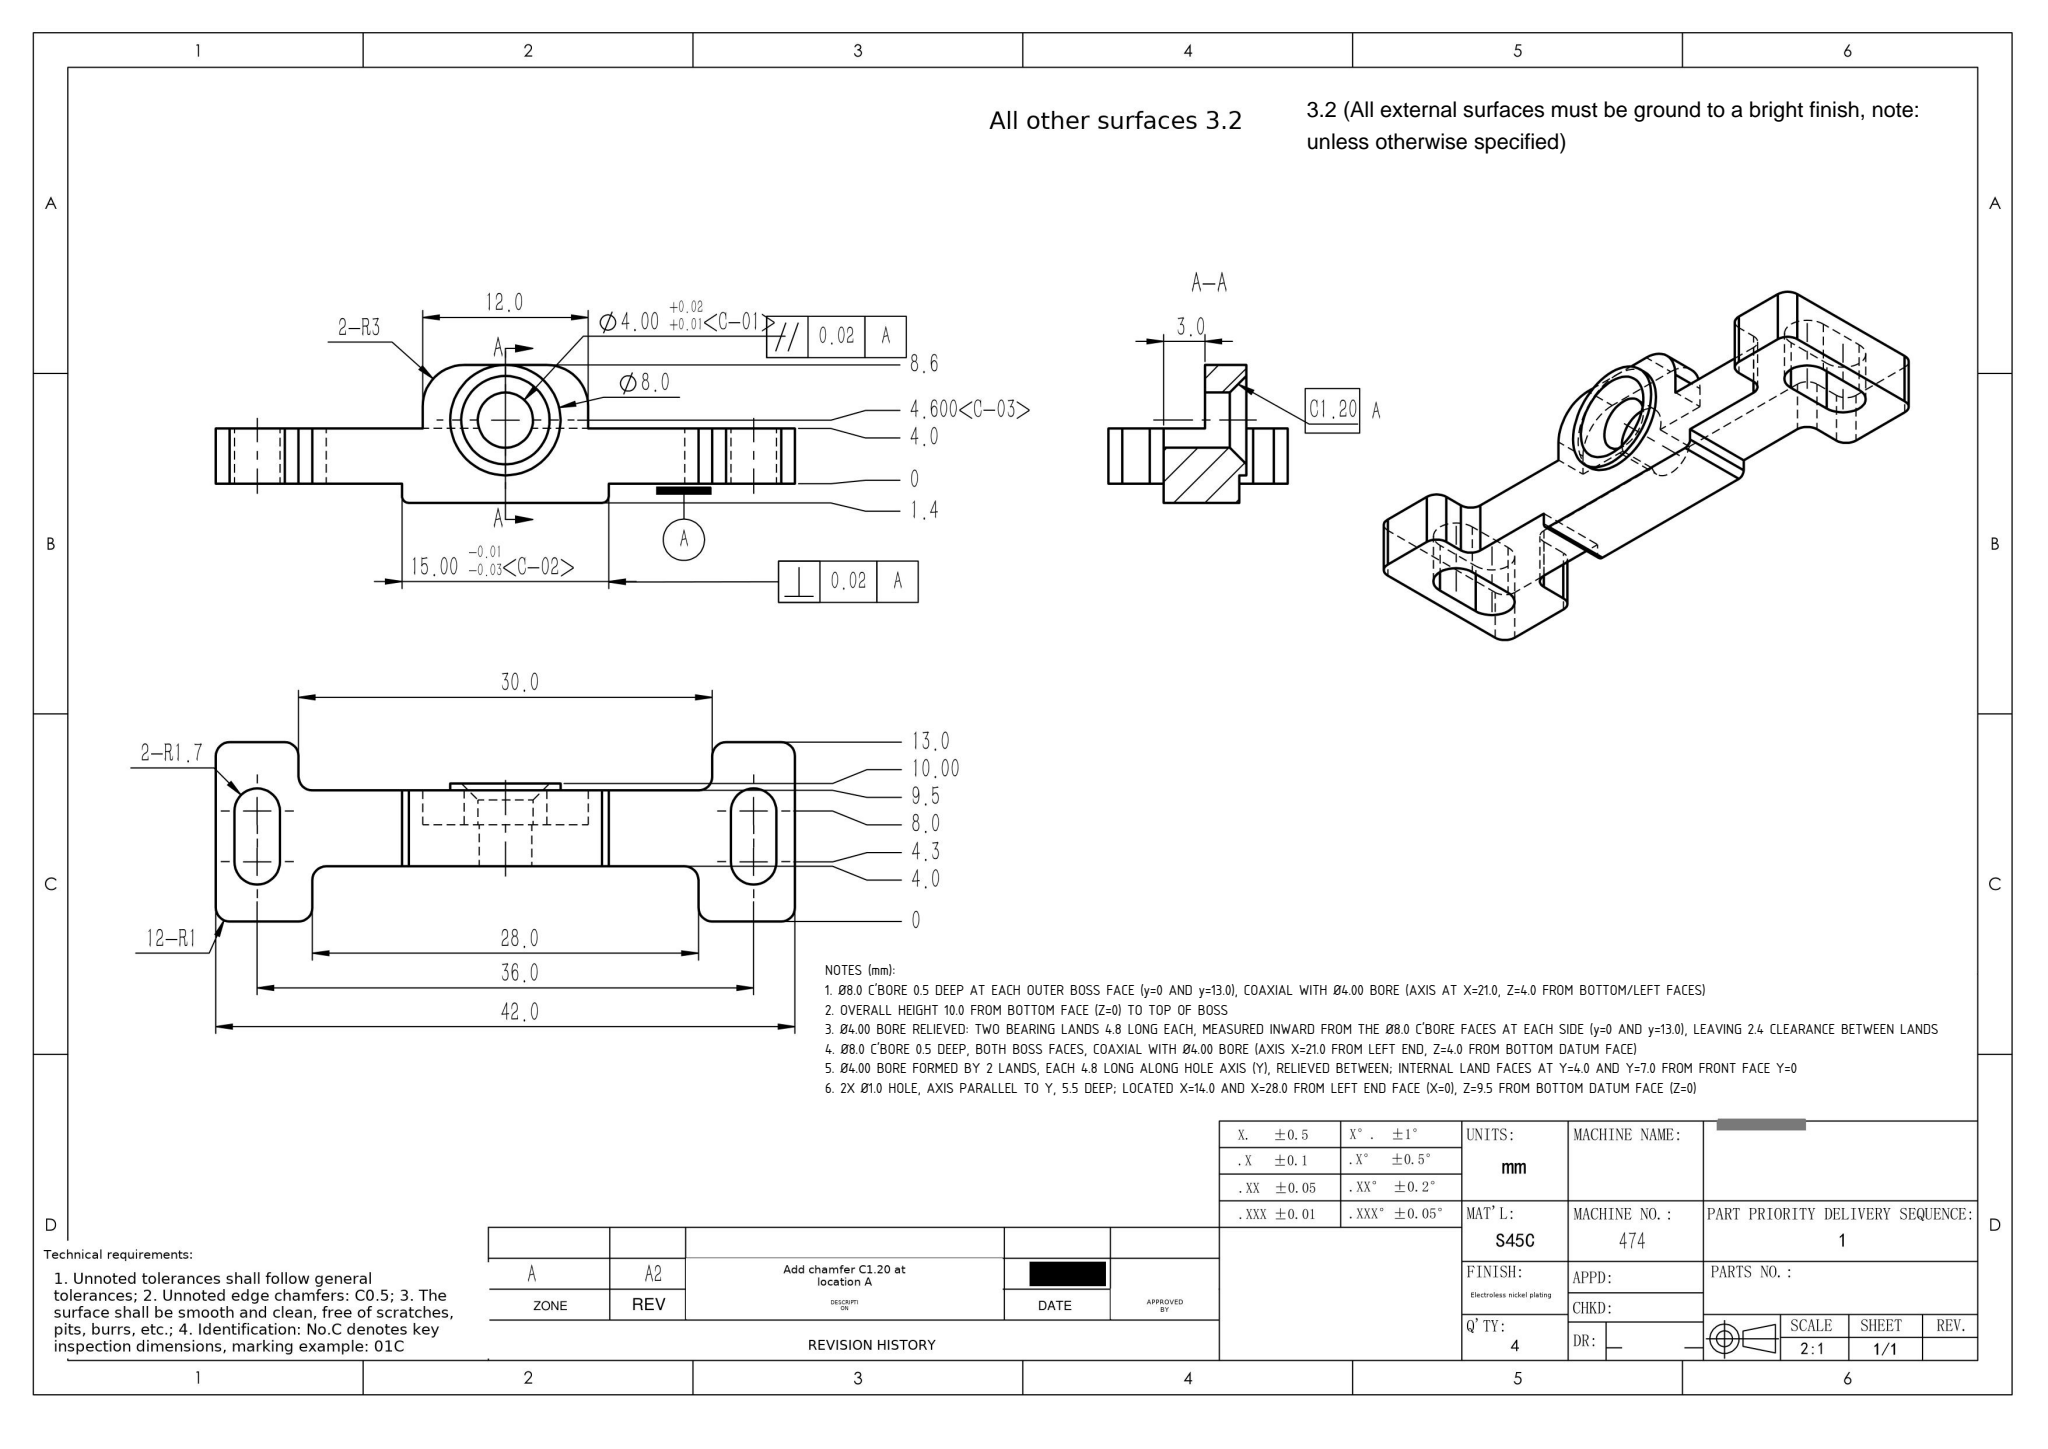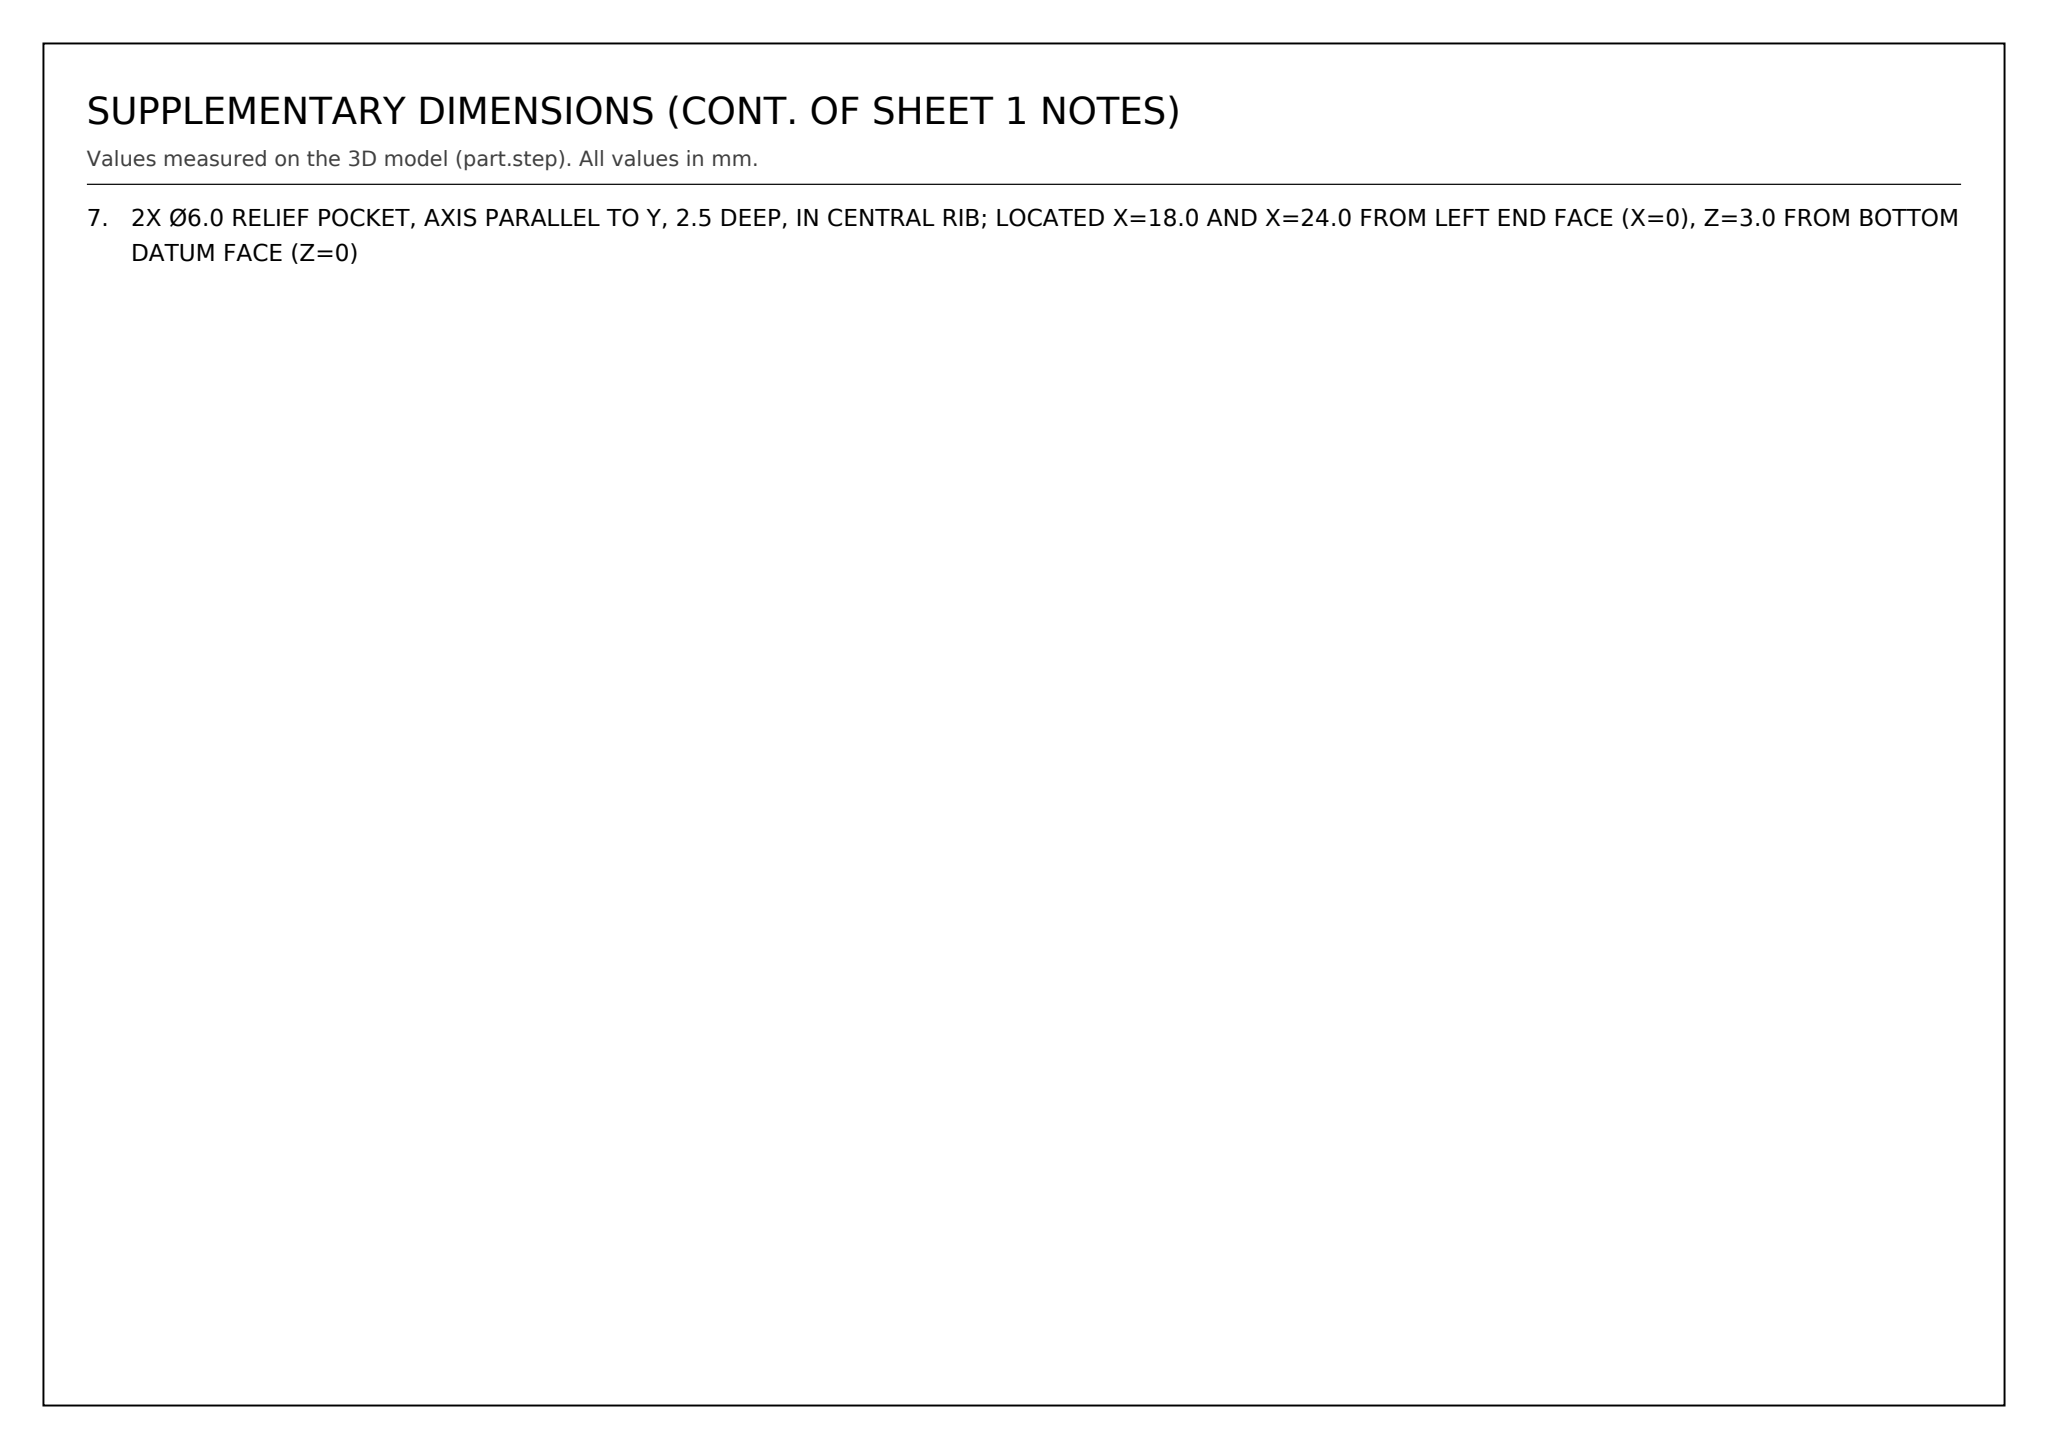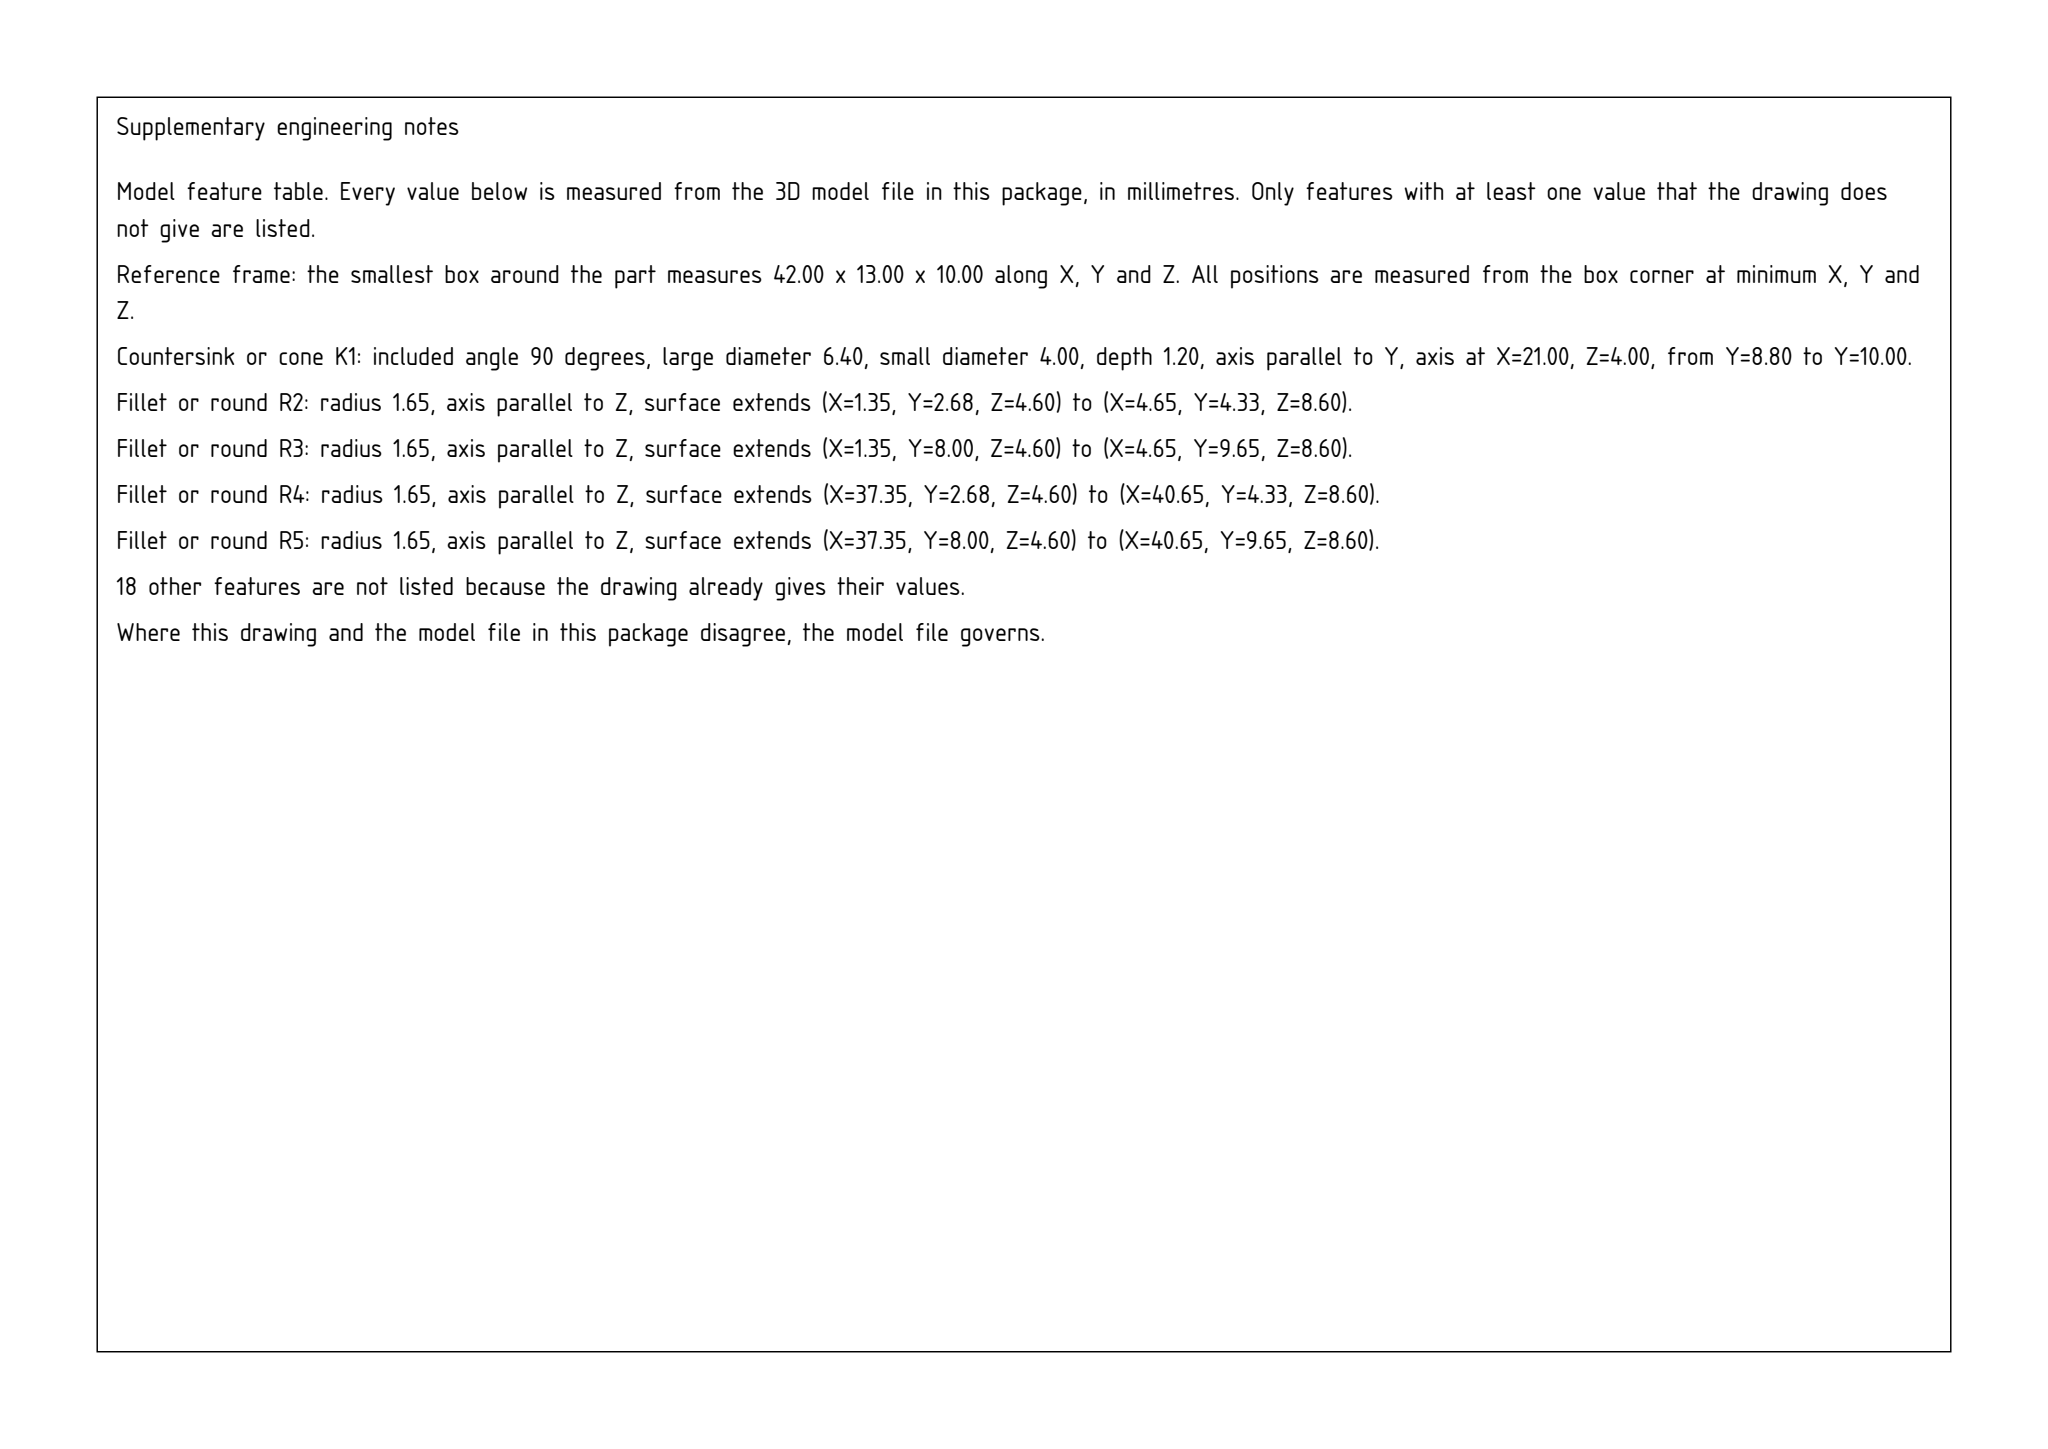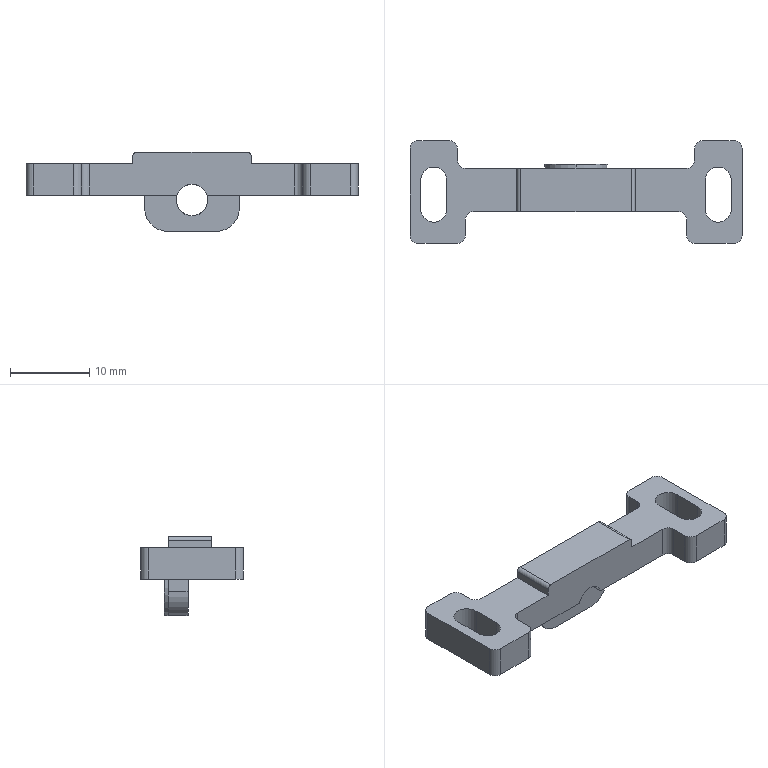Part | SolidWorks | mm | 1 solid | 54 faces | box 42 x 13 x 10 mm | volume 1355 mm3 | plane 28 | cylinder 24 | cone 2 | commonest cylinder face diameters 2 x12 3.3 x4 8 x2 4 x2 6 x2 1 x2
Drawing notes:
Ø8.0 C'BORE 0.5 DEEP AT EACH OUTER BOSS FACE (y=0 AND y=13.0), COAXIAL WITH Ø4.00 BORE (AXIS AT X=21.0, Z=4.0 FROM BOTTOM/LEFT FACES) | from the solid: cylinders: [8.0,"y",[21.0,null,4.0],0.5,count 2]
OVERALL HEIGHT 10.0 FROM BOTTOM FACE (Z=0) TO TOP OF BOSS | from the solid: bbox_xyz z = 10.0; axis_plane ["z",10.0]
Ø4.00 BORE RELIEVED: TWO BEARING LANDS 4.8 LONG EACH, MEASURED INWARD FROM THE Ø8.0 C'BORE FACES AT EACH SIDE (y=0 AND y=13.0), LEAVING 2.4 CLEARANCE BETWEEN LANDS | from the solid: cylinders: [4.0,"y",[21.0,null,4.0],4.8,count 2] with bbox y = 13.0 and 8.0 c'bore 0.5 deep each side
Ø8.0 C'BORE 0.5 DEEP, BOTH BOSS FACES, COAXIAL WITH Ø4.00 BORE (AXIS X=21.0 FROM LEFT END, Z=4.0 FROM BOTTOM DATUM FACE) | from the solid: cylinders: [8.0,"y",[21.0,null,4.0],0.5,count 2]
Ø4.00 BORE FORMED BY 2 LANDS, EACH 4.8 LONG ALONG HOLE AXIS (Y), RELIEVED BETWEEN; INTERNAL LAND FACES AT Y=4.0 AND Y=7.0 FROM FRONT FACE Y=0 | from the solid: cylinders: [4.0,"y",[21.0,null,4.0],4.8,count 2]; axis_planes ["y",4.0] and ["y",7.0]
2X Ø1.0 HOLE, AXIS PARALLEL TO Y, 5.5 DEEP; LOCATED X=14.0 AND X=28.0 FROM LEFT END FACE (X=0), Z=9.5 FROM BOTTOM DATUM FACE (Z=0) | from the solid: cylinders [1.0,"y",[14.0,null,9.5],5.5] and [1.0,"y",[28.0,null,9.5],5.5]
2X Ø6.0 RELIEF POCKET, AXIS PARALLEL TO Y, 2.5 DEEP, IN CENTRAL RIB; LOCATED X=18.0 AND X=24.0 FROM LEFT END FACE (X=0), Z=3.0 FROM BOTTOM DATUM FACE (Z=0) | from the solid: cylinders [6.0,"y",[18.0,null,3.0],2.5] and [6.0,"y",[24.0,null,3.0],2.5]
build123d program:
from build123d import *

# Parameters (mm, degrees)
SKETCH1_W           = 42
SKETCH1_H           = 7
BOSS_EXTRUDE1_DEPTH = 5
SKETCH3_W           = 13.5
SKETCH3_H           = 1.4
CUT_EXTRUDE1_DEPTH  = 7
SKETCH4_W           = 15
SKETCH4_H           = 4.6
CUT_EXTRUDE2_DEPTH  = 7
SKETCH5_R           = 2
CUT_EXTRUDE3_DEPTH  = 7
FILLET1_R           = 3
SKETCH6_W           = 9
SKETCH6_H           = 0.5
CUT_EXTRUDE4_DEPTH  = 10
FILLET2_R           = 3
SKETCH8_W           = 6
SKETCH8_H           = 4
BOSS_EXTRUDE2_DEPTH = 3
SKETCH11_W          = 7
SKETCH11_H          = 3
BOSS_EXTRUDE3_DEPTH = 4
CUT_EXTRUDE5_DEPTH  = 24.878
FILLET4_R           = 0.5
FILLET5_R           = 1
SKETCH12_W          = 12
SKETCH12_H          = 4.6
CUT_EXTRUDE6_DEPTH  = 4
SKETCH14_R          = 10
SKETCH14_R_2        = 4
CUT_EXTRUDE7_DEPTH  = 0.5
CUT_EXTRUDE8_DEPTH  = 24.878
CHAMFER2_SIZE       = 1.2


with BuildPart() as part:
    # Sketch1 → Boss-Extrude1 (new, symmetric)
    with BuildSketch(Plane.XY):
        with Locations((0, 3.5)):
            Rectangle(SKETCH1_W, SKETCH1_H)
    extrude(amount=BOSS_EXTRUDE1_DEPTH, both=True)

    # Sketch3 → Cut-Extrude1 (cut)
    with BuildSketch(Plane.XZ):
        with Locations((-14.25, 4.3)):
            Rectangle(SKETCH3_W, SKETCH3_H)
        with Locations((14.25, 4.3)):
            Rectangle(SKETCH3_W, SKETCH3_H)
    extrude(amount=-CUT_EXTRUDE1_DEPTH, mode=Mode.SUBTRACT)

    # Sketch4 → Cut-Extrude2 (cut)
    with BuildSketch(Plane.XZ):
        with Locations((-13.5, -2.7)):
            Rectangle(SKETCH4_W, SKETCH4_H)
        with Locations((13.5, -2.7)):
            Rectangle(SKETCH4_W, SKETCH4_H)
    extrude(amount=-CUT_EXTRUDE2_DEPTH, mode=Mode.SUBTRACT)

    # Sketch5 → Cut-Extrude3 (cut)
    with BuildSketch(Plane.XZ):
        with Locations(Location((0, -1, 0), (0, 0, 270))):
            Circle(SKETCH5_R)
    extrude(amount=-CUT_EXTRUDE3_DEPTH, mode=Mode.SUBTRACT)

    # Fillet1
    fillet1_edges = [part.edges().sort_by_distance(p)[0] for p in [
        (-6, 3.5, -5),
        (6, 3.5, -5),
    ]]
    fillet(fillet1_edges, radius=FILLET1_R)

    # Sketch6 → Cut-Extrude4 (cut)
    with BuildSketch(Plane.XY.offset(5)):
        with Locations((-10.5, 6.75)):
            Rectangle(SKETCH6_W, SKETCH6_H)
        with Locations((10.5, 6.75)):
            Rectangle(SKETCH6_W, SKETCH6_H)
    extrude(amount=-CUT_EXTRUDE4_DEPTH, mode=Mode.SUBTRACT)

    # Fillet2
    fillet2_edges = [part.edges().sort_by_distance(p)[0] for p in [
        (6, 6.75, 5),
        (-6, 6.75, 5),
    ]]
    fillet(fillet2_edges, radius=FILLET2_R)

    # Sketch8 → Boss-Extrude2 (add)
    with BuildSketch(Plane(origin=(0, 7, 0), x_dir=(1, 0, 0), z_dir=(0, 1, 0))):
        with Locations((-18, -1.6)):
            Rectangle(SKETCH8_W, SKETCH8_H)
        with Locations((18, -1.6)):
            Rectangle(SKETCH8_W, SKETCH8_H)
    extrude(amount=BOSS_EXTRUDE2_DEPTH)

    # Sketch11 → Boss-Extrude3 (add)
    with BuildSketch(Plane(origin=(0, 0, -0.4), x_dir=(-1, 0, 0), z_dir=(0, 0, -1))):
        with Locations((-17.5, -1.5)):
            Rectangle(SKETCH11_W, SKETCH11_H)
        with Locations((17.5, -1.5)):
            Rectangle(SKETCH11_W, SKETCH11_H)
    extrude(amount=-BOSS_EXTRUDE3_DEPTH)

    # Sketch9 → Cut-Extrude5 (cut, through all)
    with BuildSketch(Plane(origin=(0, 0, -0.4), x_dir=(-1, 0, 0), z_dir=(0, 0, -1))):
        with BuildLine():
            Line((-19.65, 5), (-19.65, 1.33))
            ThreePointArc((-19.65, 1.33), (-18, -0.32), (-16.35, 1.33))
            Line((-16.35, 1.33), (-16.35, 5))
            ThreePointArc((-16.35, 5), (-18, 6.65), (-19.65, 5))
        make_face()
        with BuildLine():
            Line((16.35, 5), (16.35, 1.33))
            ThreePointArc((16.35, 1.33), (18, -0.32), (19.65, 1.33))
            Line((19.65, 1.33), (19.65, 5))
            ThreePointArc((19.65, 5), (18, 6.65), (16.35, 5))
        make_face()
    extrude(amount=-CUT_EXTRUDE5_DEPTH, mode=Mode.SUBTRACT)

    # Fillet4
    fillet4_edges = [part.edges().sort_by_distance(p)[0] for p in [
        (7.5, 3.25, 5),
        (-7.5, 3.25, 5),
    ]]
    fillet(fillet4_edges, radius=FILLET4_R)

    # Fillet5
    fillet5_edges = [part.edges().sort_by_distance(p)[0] for p in [
        (-15, 6.5, 1.6),
        (-15, 10, 1.6),
        (-21, 10, 1.6),
        (-21, -3, 1.6),
        (-14, -3, 1.6),
        (-14, 0, 1.6),
        (15, 6.5, 1.6),
        (15, 10, 1.6),
        (21, 10, 1.6),
        (21, -3, 1.6),
        (14, -3, 1.6),
        (14, 0, 1.6),
    ]]
    fillet(fillet5_edges, radius=FILLET5_R)

    # Sketch12 → Cut-Extrude6 (cut)
    with BuildSketch(Plane.XZ):
        with Locations((0, -2.7)):
            Rectangle(SKETCH12_W, SKETCH12_H)
    extrude(amount=-CUT_EXTRUDE6_DEPTH, mode=Mode.SUBTRACT)

    # Sketch14 → Cut-Extrude7 (cut)
    with BuildSketch(Plane(origin=(0, 7, 0), x_dir=(1, 0, 0), z_dir=(0, 1, 0))):
        with Locations((0, 1)):
            Circle(SKETCH14_R)
        with Locations(Location((0, 1, 0), (0, 0, 270))):
            Circle(SKETCH14_R_2, mode=Mode.SUBTRACT)
    extrude(amount=-CUT_EXTRUDE7_DEPTH, mode=Mode.SUBTRACT)

    # Sketch15 → Cut-Extrude8 (cut, through all)
    with BuildSketch(Plane(origin=(0, 0, -0.4), x_dir=(-1, 0, 0), z_dir=(0, 0, -1))):
        with BuildLine():
            Line((-14, -1), (-14, -3))
            Line((-14, -3), (14, -3))
            Line((14, -3), (14, -1))
            Line((14, -1), (14, 0))
            ThreePointArc((14, 0), (13.707, 0.7071), (13, 1))
            Line((13, 1), (1.908, 1))
            Line((1.908, 1), (-1.908, 1))
            Line((-1.908, 1), (-13, 1))
            ThreePointArc((-13, 1), (-13.707, 0.7071), (-14, 0))
            Line((-14, 0), (-14, -1))
        make_face()
    extrude(amount=-CUT_EXTRUDE8_DEPTH, mode=Mode.SUBTRACT)

    # Chamfer2
    chamfer2_edges = [part.edges().sort_by_distance(p)[0] for p in [
        (0, 7, 1),
    ]]
    chamfer(chamfer2_edges, length=CHAMFER2_SIZE)


solid = part.part